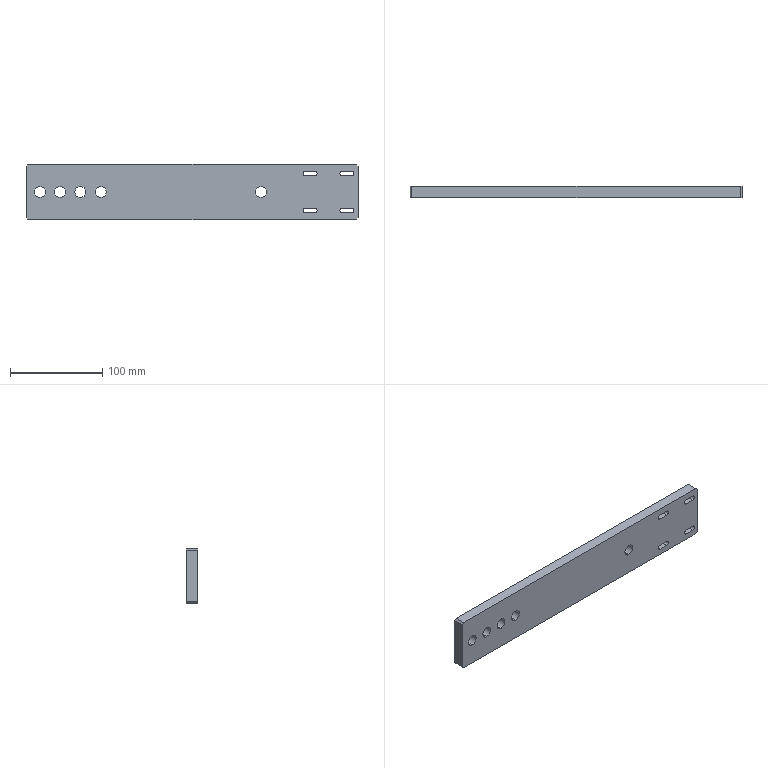Component | SolidWorks | Part41-1 | 1 solid | 56 faces | volume 246356 mm3 | plane 30 | cylinder 26 | commonest cylinder face diameters 12 x10 5.3 x8 10 x8